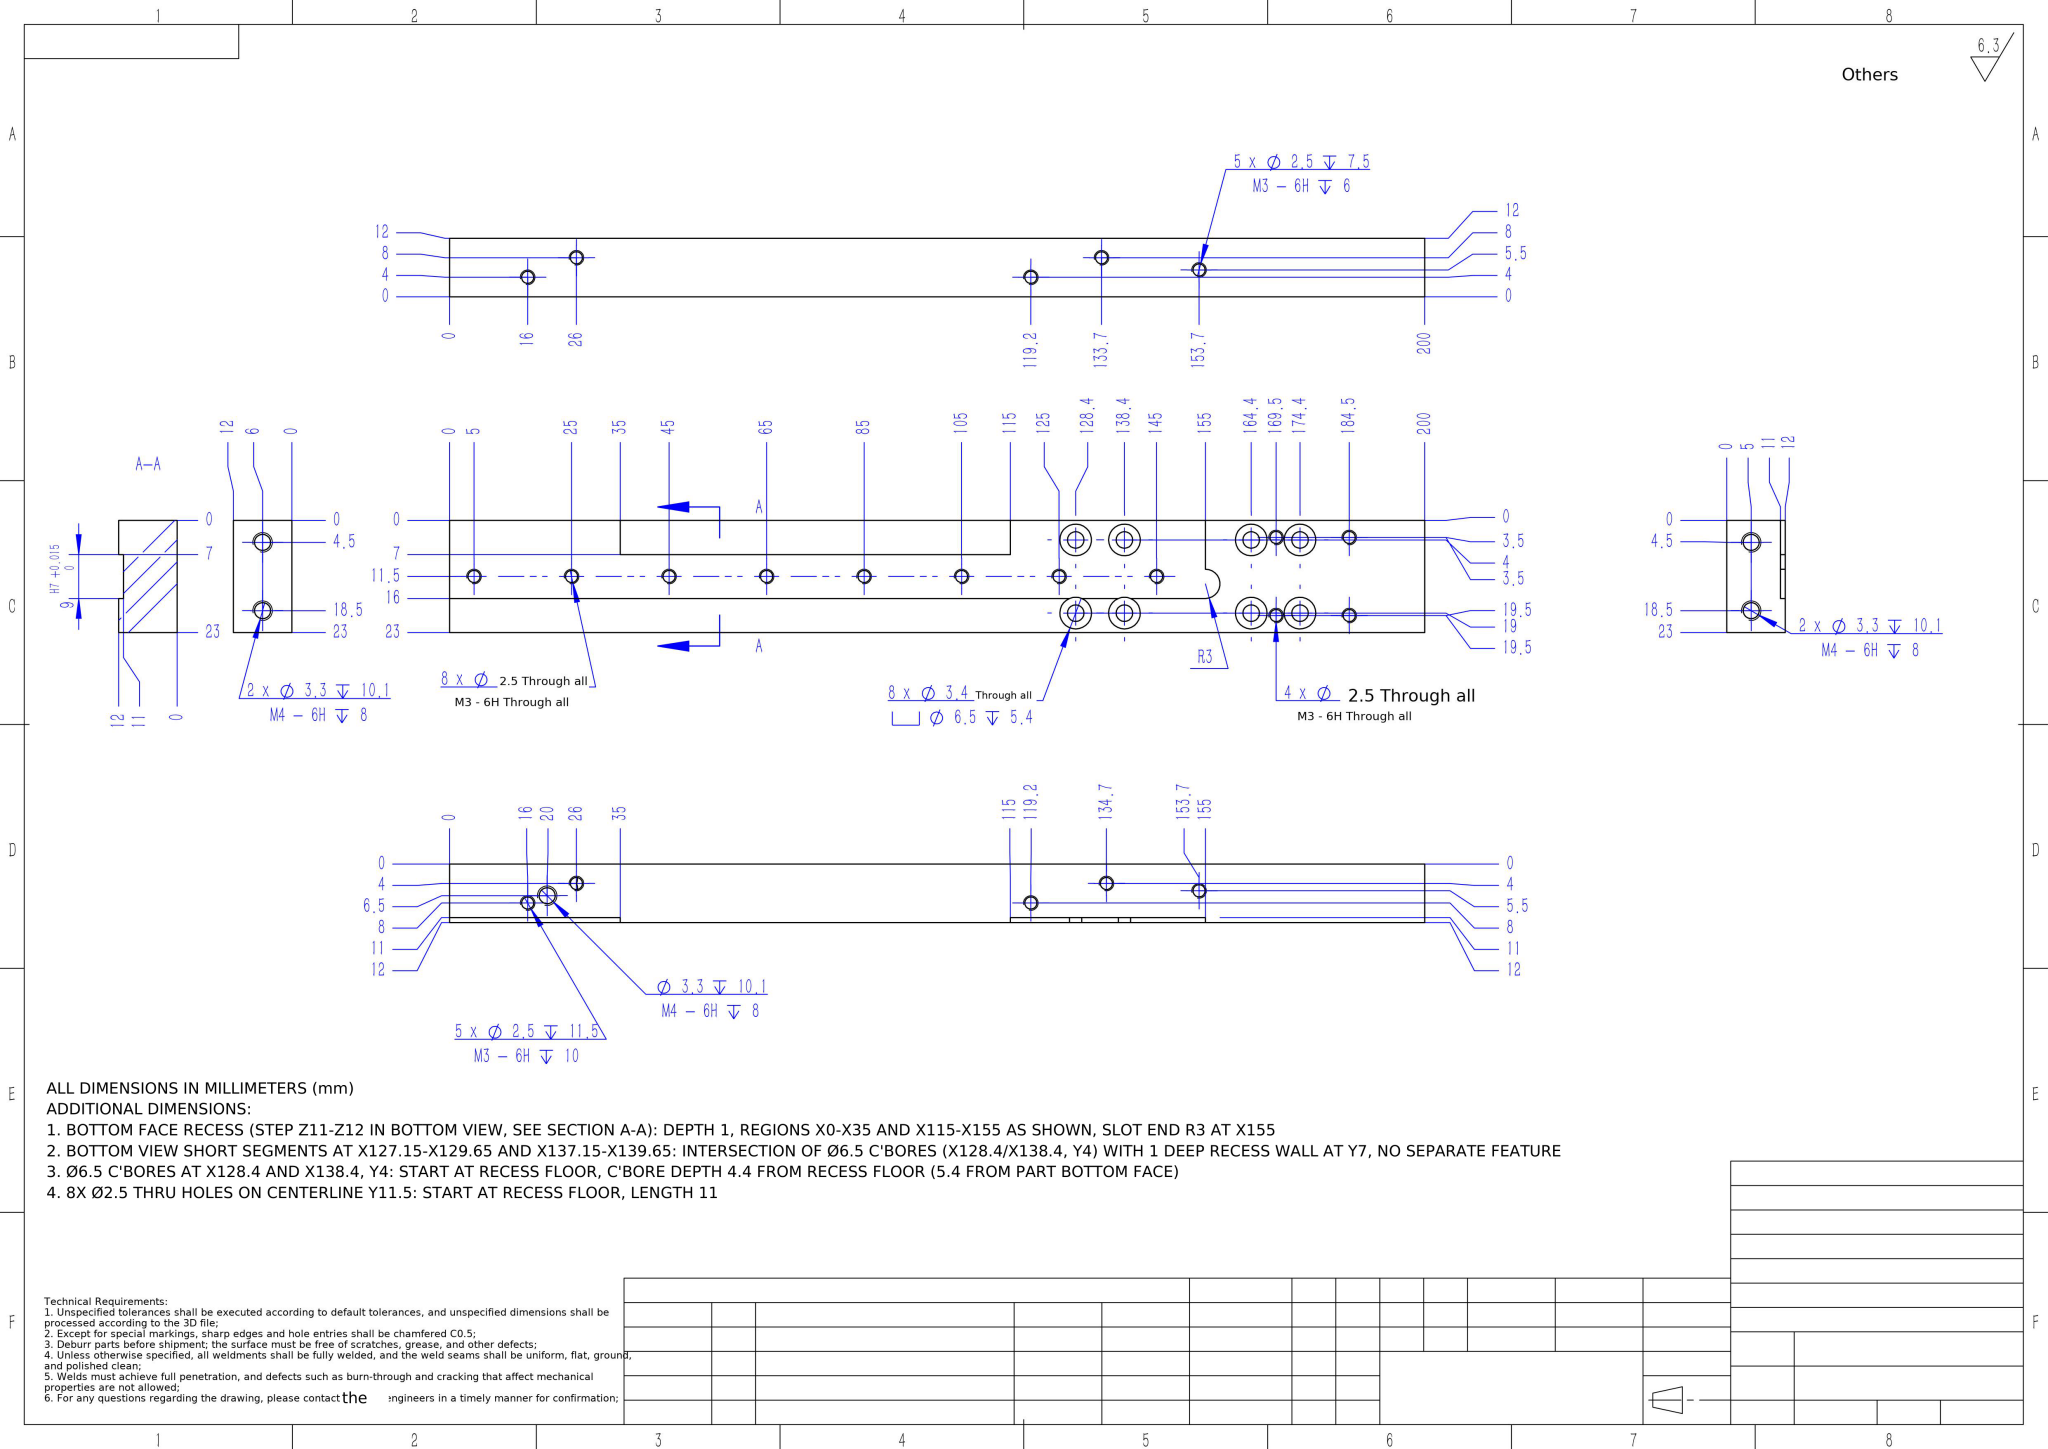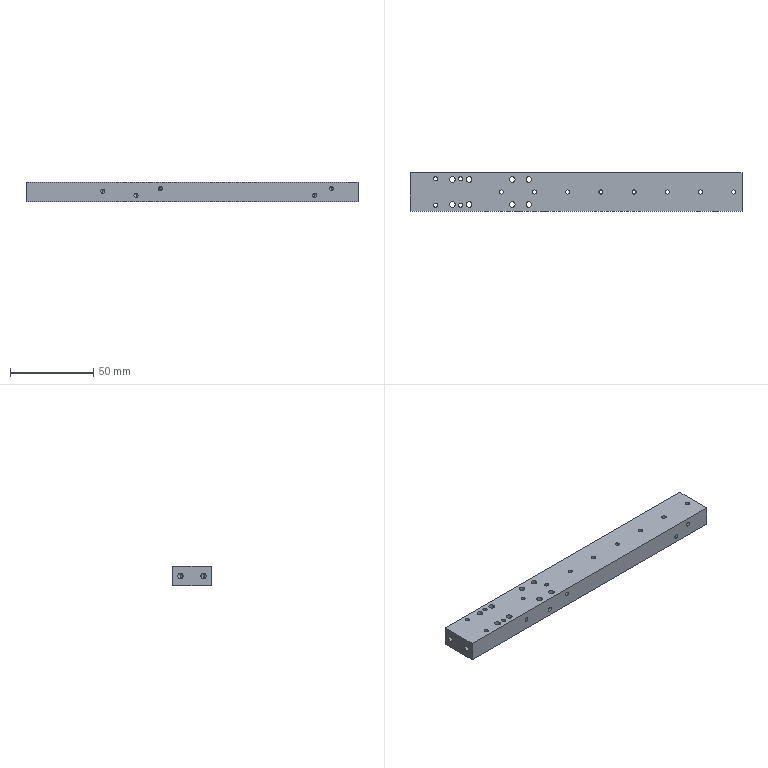Part | NX | mm | 1 solid | 141 faces | box 200 x 23 x 12 mm | volume 49832 mm3 | cylinder 88 | cone 30 | plane 23 | commonest cylinder face diameters 2.5 x44 6.5 x16 3.4 x16 3.3 x10 6 x2